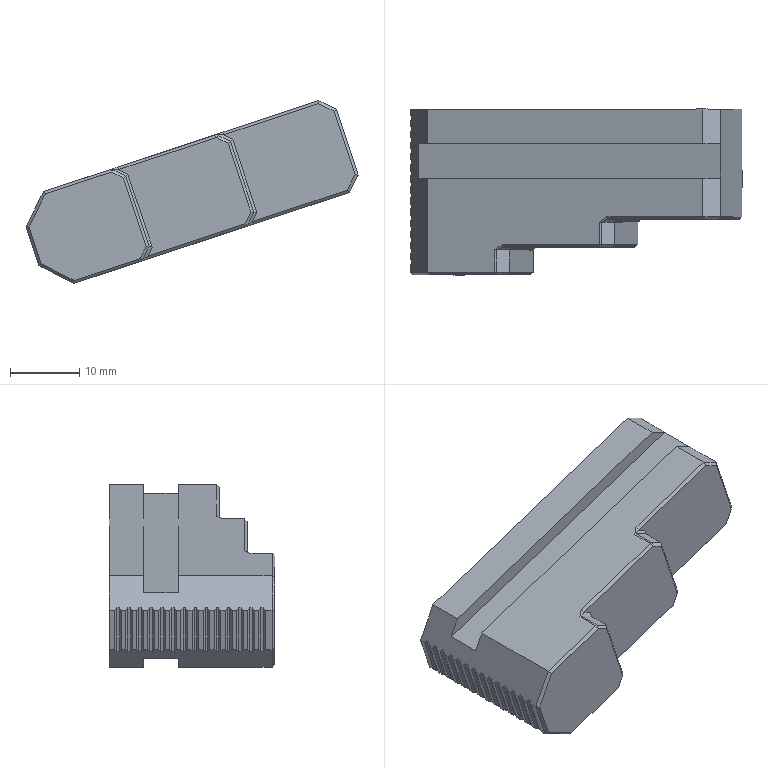Component | SolidWorks | HZ022-Three-JawChuckJaw-1 | 1 solid | 120 faces | volume 12064 mm3 | plane 116 | spline 4